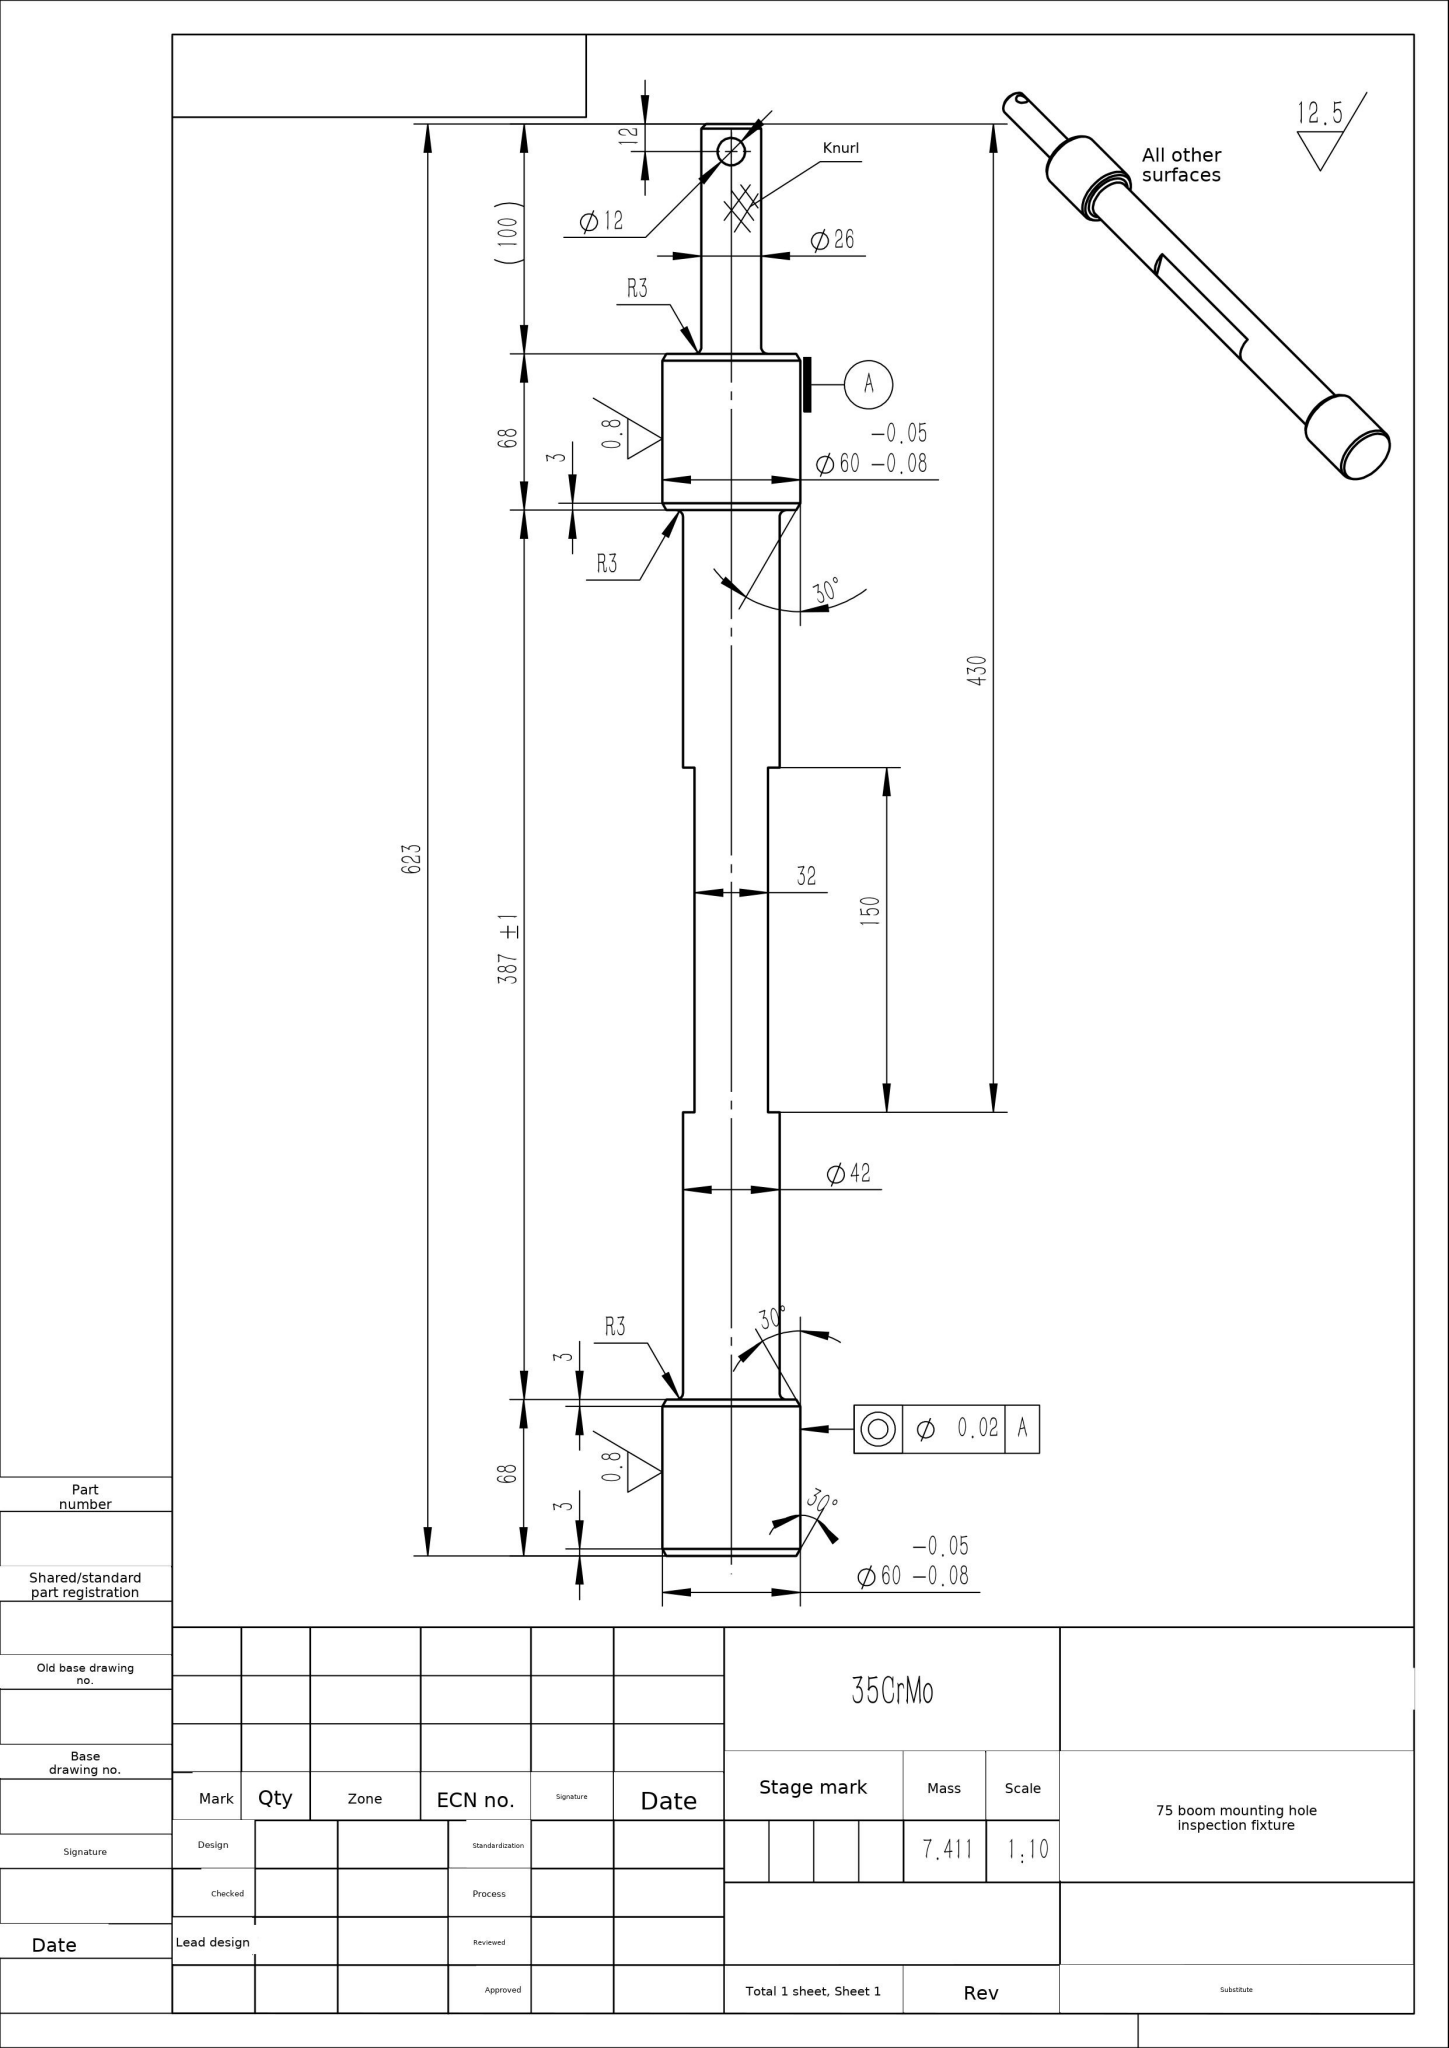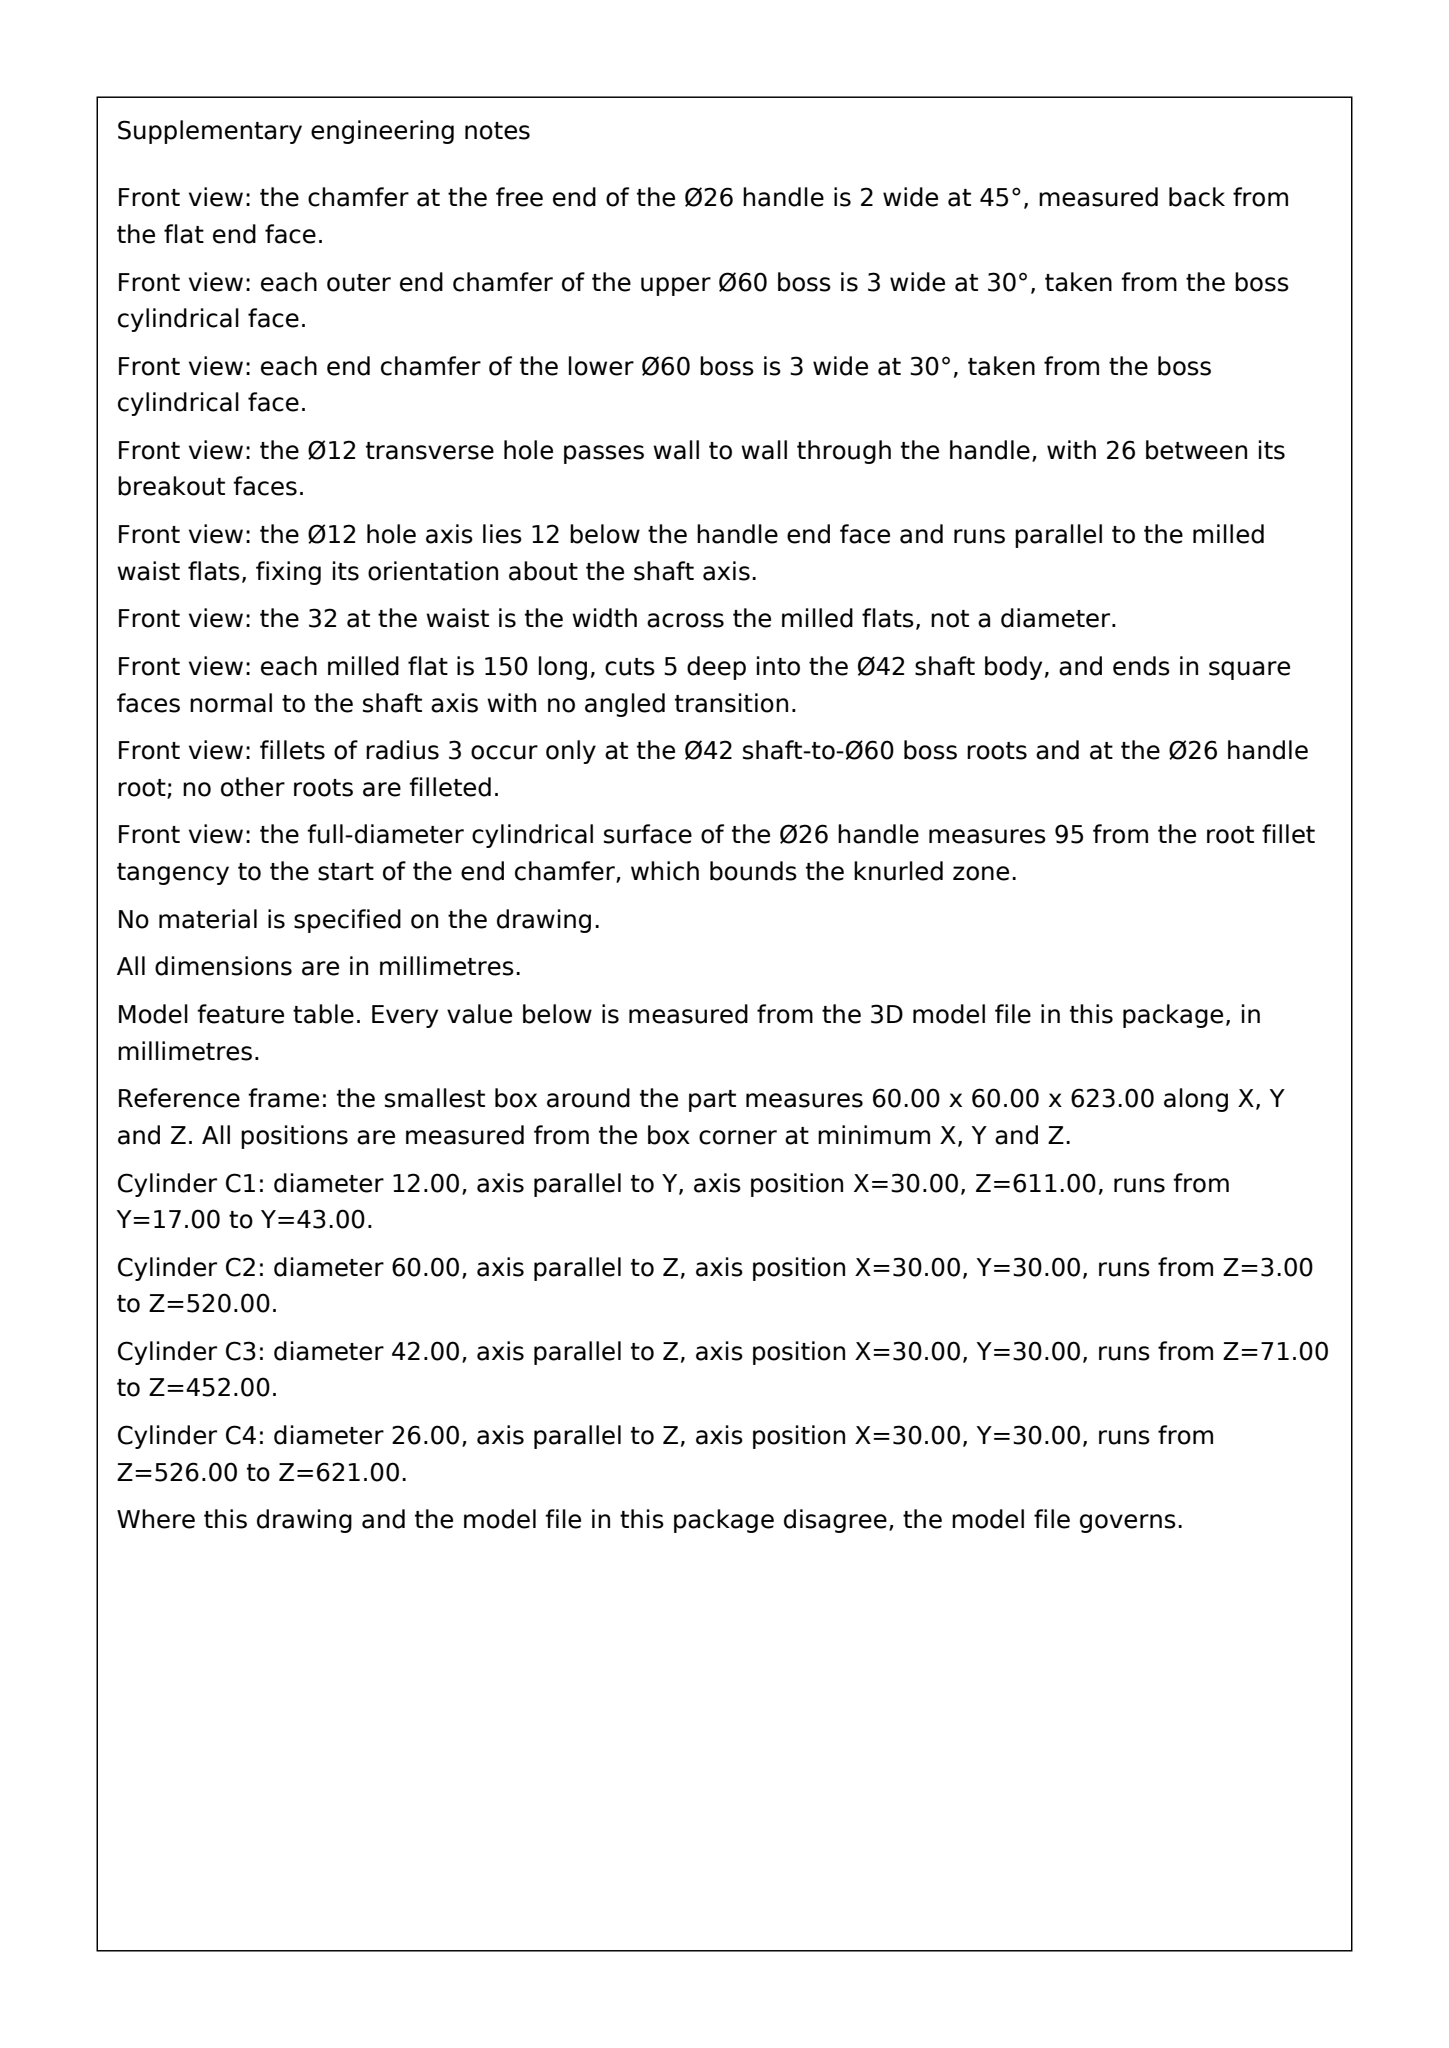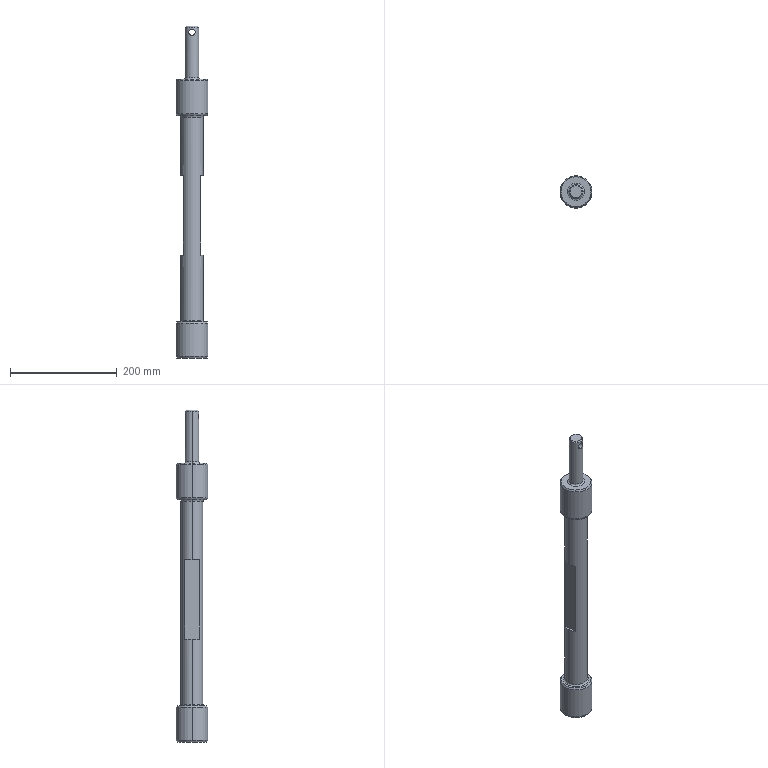Part | SolidWorks | mm | 1 solid | 37 faces | box 60 x 60 x 623 mm | volume 941621 mm3 | plane 11 | cylinder 10 | cone 10 | torus 6 | commonest cylinder face diameters 60 x4 12 x2 26 x2 42 x2
Drawing notes:
Ø26 SHAFT TOP END: C2 X 45° TO Ø22 | from the solid: cone incl 90°, ref dia 22.0, from z=621 to 623 on Ø26 shaft (z 526-621); top face z=623 extent Ø22
UPPER END TOP Ø60 BOSS: 3 X 30° CHAM, TYP BOTH BOSS ENDS | from the solid: cone incl 60° (30° per side) at z=520-523, ref dia 56.54; Ø60 boss z=458-520, face z=523
build123d program:
from build123d import *

# Parameters (mm, degrees)
SKETCH1_R               = 30
BOSS_EXTRUDE1_DEPTH     = 68
CHAMFER1_SIZE           = 3
CHAMFER1_SIZE2          = 1.732
CHAMFER2_SIZE           = 3
CHAMFER2_SIZE2          = 1.732
SKETCH2_R               = 21
BOSS_EXTRUDE2_DEPTH     = 387
BOSS_EXTRUDE3_START     = 68
SKETCH3_R               = 30
BOSS_EXTRUDE3_DEPTH     = 68
CHAMFER3_SIZE           = 3
CHAMFER3_SIZE2          = 1.732
CHAMFER4_SIZE           = 3
CHAMFER4_SIZE2          = 1.732
SKETCH4_R               = 13
BOSS_EXTRUDE4_DEPTH     = 100
CHAMFER5_SIZE           = 2
CUT_EXTRUDE1_DEPTH      = 457.974
CUT_EXTRUDE1_DEPTH_BACK = 457.974
SKETCH5_R               = 6
FILLET2_R               = 3
FILLET3_R               = 3
CUT_EXTRUDE2_DEPTH      = 457.974
CUT_EXTRUDE2_DEPTH_BACK = 457.974
SKETCH6_W               = 72.349
SKETCH6_H               = 150
SKETCH6_W_2             = 83.674


with BuildPart() as part:
    # Sketch1 → Boss-Extrude1 (new body)
    with BuildSketch(Plane.XY):
        Circle(SKETCH1_R)
    extrude(amount=BOSS_EXTRUDE1_DEPTH)

    # Chamfer1
    chamfer1_edges = [part.edges().sort_by_distance(p)[0] for p in [
        (-30, 0, 68),
    ]]
    chamfer1_side = [part.faces().sort_by_distance(p)[0] for p in [
        (-30, 0, 34),
    ]]
    chamfer(chamfer1_edges, length=CHAMFER1_SIZE, length2=CHAMFER1_SIZE2, reference=chamfer1_side[0])

    # Chamfer2
    chamfer2_edges = [part.edges().sort_by_distance(p)[0] for p in [
        (-30, 0, 0),
    ]]
    chamfer2_side = [part.faces().sort_by_distance(p)[0] for p in [
        (-30, 0, 32.5),
    ]]
    chamfer(chamfer2_edges, length=CHAMFER2_SIZE, length2=CHAMFER2_SIZE2, reference=chamfer2_side[0])

    # Sketch2 → Boss-Extrude2 (add)
    with BuildSketch(Plane(origin=(0, 0, 0), x_dir=(-1, 0, 0), z_dir=(0, 0, -1))):
        with Locations(Location((0, 0, 0), (0, 0, 180))):
            Circle(SKETCH2_R)
    extrude(amount=BOSS_EXTRUDE2_DEPTH)

    # Sketch3 → Boss-Extrude3 (add)
    with BuildSketch(Plane(origin=(0, 0, -387), x_dir=(-1, 0, 0), z_dir=(0, 0, -1)).offset(BOSS_EXTRUDE3_START)):
        with Locations(Location((0, 0, 0), (0, 0, 180))):
            Circle(SKETCH3_R)
    extrude(amount=-BOSS_EXTRUDE3_DEPTH)

    # Chamfer3
    chamfer3_edges = [part.edges().sort_by_distance(p)[0] for p in [
        (-30, 0, -387),
    ]]
    chamfer3_side = [part.faces().sort_by_distance(p)[0] for p in [
        (-30, 0, -421),
    ]]
    chamfer(chamfer3_edges, length=CHAMFER3_SIZE, length2=CHAMFER3_SIZE2, reference=chamfer3_side[0])

    # Chamfer4
    chamfer4_edges = [part.edges().sort_by_distance(p)[0] for p in [
        (-30, 0, -455),
    ]]
    chamfer4_side = [part.faces().sort_by_distance(p)[0] for p in [
        (-30, 0, -422.5),
    ]]
    chamfer(chamfer4_edges, length=CHAMFER4_SIZE, length2=CHAMFER4_SIZE2, reference=chamfer4_side[0])

    # Sketch4 → Boss-Extrude4 (add)
    with BuildSketch(Plane.XY.offset(68)):
        Circle(SKETCH4_R)
    extrude(amount=BOSS_EXTRUDE4_DEPTH)

    # Chamfer5
    chamfer5_edges = [part.edges().sort_by_distance(p)[0] for p in [
        (-13, 0, 168),
    ]]
    chamfer(chamfer5_edges, length=CHAMFER5_SIZE)

    # Sketch5 → Cut-Extrude1 (cut, two sides: drawn at the far end of the back side and taken through both)
    with BuildSketch(Plane(origin=(0, 0, 0), x_dir=(1, 0, 0), z_dir=(0, 1, 0)).offset(-CUT_EXTRUDE1_DEPTH_BACK)):
        with Locations(Location((0, -156, 0), (0, 0, 270))):
            Circle(SKETCH5_R)
    extrude(amount=CUT_EXTRUDE1_DEPTH + CUT_EXTRUDE1_DEPTH_BACK, mode=Mode.SUBTRACT)

    # Fillet2
    fillet2_edges = [part.edges().sort_by_distance(p)[0] for p in [
        (-13, 0, 68),
    ]]
    fillet(fillet2_edges, radius=FILLET2_R)

    # Fillet3
    fillet3_edges = [part.edges().sort_by_distance(p)[0] for p in [
        (-21, 0, 0),
        (-21, 0, -387),
    ]]
    fillet(fillet3_edges, radius=FILLET3_R)

    # Sketch6 → Cut-Extrude2 (cut, two sides: drawn at the far end of the back side and taken through both)
    with BuildSketch(Plane(origin=(0, 0, 0), x_dir=(1, 0, 0), z_dir=(0, 1, 0)).offset(-CUT_EXTRUDE2_DEPTH_BACK)):
        with Locations((52.175, 187)):
            Rectangle(SKETCH6_W, SKETCH6_H)
        with Locations((-57.837, 187)):
            Rectangle(SKETCH6_W_2, SKETCH6_H)
    extrude(amount=CUT_EXTRUDE2_DEPTH + CUT_EXTRUDE2_DEPTH_BACK, mode=Mode.SUBTRACT)


solid = part.part